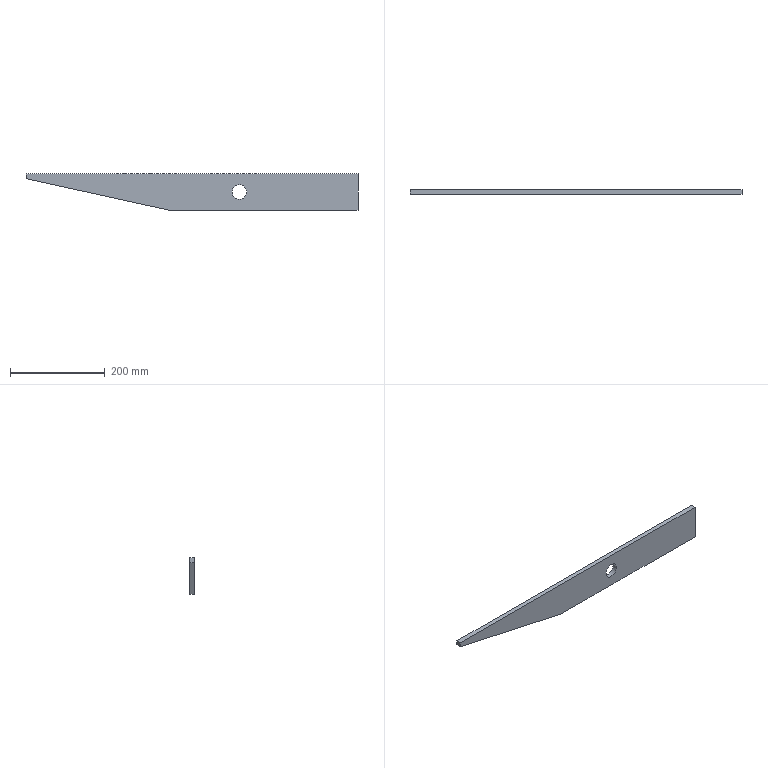Component | NX | CHAPA_FUNDO | 1 solid | 8 faces | box 700 x 10 x 76.2 mm | volume 426852 mm3 | plane 7 | cylinder 1 | commonest cylinder face diameters 31 x1
STEP:
#1=CARTESIAN_POINT('',(0.,0.,0.));
#2=DIRECTION('',(0.,0.,1.));
#3=DIRECTION('',(1.,0.,0.));
#4=AXIS2_PLACEMENT_3D('',#1,#2,#3);
#5=CARTESIAN_POINT('',(-60.,5.2,80.));
#6=VERTEX_POINT('',#5);
#7=CARTESIAN_POINT('',(-60.,5.2,3.8));
#8=VERTEX_POINT('',#7);
#9=CARTESIAN_POINT('',(-60.,5.2,80.));
#10=DIRECTION('',(-0.,0.,-1.));
#11=VECTOR('',#10,1.);
#12=LINE('',#9,#11);
#13=CARTESIAN_POINT('',(-60.,15.2,80.));
#14=DIRECTION('',(-1.,0.,0.));
#15=DIRECTION('',(-0.,0.,-1.));
#16=AXIS2_PLACEMENT_3D('',#13,#14,#15);
#17=PLANE('',#16);
#18=CARTESIAN_POINT('',(0.,10.));
#19=DIRECTION('',(1.,0.));
#20=VECTOR('',#19,1.);
#21=LINE('',#18,#20);
#22=(GEOMETRIC_REPRESENTATION_CONTEXT(2)PARAMETRIC_REPRESENTATION_CONTEXT()REPRESENTATION_CONTEXT('',''));
#23=DEFINITIONAL_REPRESENTATION('',(#21),#22);
#24=PCURVE('',#17,#23);
#25=CARTESIAN_POINT('',(-310.,5.2,41.9));
#26=DIRECTION('',(0.,1.,0.));
#27=DIRECTION('',(0.,0.,-1.));
#28=AXIS2_PLACEMENT_3D('',#25,#26,#27);
#29=PLANE('',#28);
#30=CARTESIAN_POINT('',(-38.1,-250.));
#31=DIRECTION('',(1.,0.));
#32=VECTOR('',#31,1.);
#33=LINE('',#30,#32);
#34=(GEOMETRIC_REPRESENTATION_CONTEXT(2)PARAMETRIC_REPRESENTATION_CONTEXT()REPRESENTATION_CONTEXT('',''));
#35=DEFINITIONAL_REPRESENTATION('',(#33),#34);
#36=PCURVE('',#29,#35);
#37=SURFACE_CURVE('',#12,(#24,#36),.PCURVE_S1.);
#38=EDGE_CURVE('',#6,#8,#37,.T.);
#39=ORIENTED_EDGE('',*,*,#38,.T.);
#40=CARTESIAN_POINT('',(-60.,15.2,3.8));
#41=VERTEX_POINT('',#40);
#42=CARTESIAN_POINT('',(-60.,15.2,3.8));
#43=DIRECTION('',(0.,-1.,0.));
#44=VECTOR('',#43,1.);
#45=LINE('',#42,#44);
#46=CARTESIAN_POINT('',(76.2,0.));
#47=DIRECTION('',(0.,1.));
#48=VECTOR('',#47,1.);
#49=LINE('',#46,#48);
#50=(GEOMETRIC_REPRESENTATION_CONTEXT(2)PARAMETRIC_REPRESENTATION_CONTEXT()REPRESENTATION_CONTEXT('',''));
#51=DEFINITIONAL_REPRESENTATION('',(#49),#50);
#52=PCURVE('',#17,#51);
#53=CARTESIAN_POINT('',(-60.,15.2,3.8));
#54=DIRECTION('',(0.,0.,1.));
#55=DIRECTION('',(-1.,0.,0.));
#56=AXIS2_PLACEMENT_3D('',#53,#54,#55);
#57=PLANE('',#56);
#58=CARTESIAN_POINT('',(0.,0.));
#59=DIRECTION('',(0.,1.));
#60=VECTOR('',#59,1.);
#61=LINE('',#58,#60);
#62=(GEOMETRIC_REPRESENTATION_CONTEXT(2)PARAMETRIC_REPRESENTATION_CONTEXT()REPRESENTATION_CONTEXT('',''));
#63=DEFINITIONAL_REPRESENTATION('',(#61),#62);
#64=PCURVE('',#57,#63);
#65=SURFACE_CURVE('',#45,(#52,#64),.PCURVE_S1.);
#66=EDGE_CURVE('',#41,#8,#65,.T.);
#67=ORIENTED_EDGE('',*,*,#66,.F.);
#68=CARTESIAN_POINT('',(-60.,15.2,80.));
#69=VERTEX_POINT('',#68);
#70=CARTESIAN_POINT('',(-60.,15.2,80.));
#71=DIRECTION('',(-0.,0.,-1.));
#72=VECTOR('',#71,1.);
#73=LINE('',#70,#72);
#74=CARTESIAN_POINT('',(0.,0.));
#75=DIRECTION('',(1.,0.));
#76=VECTOR('',#75,1.);
#77=LINE('',#74,#76);
#78=(GEOMETRIC_REPRESENTATION_CONTEXT(2)PARAMETRIC_REPRESENTATION_CONTEXT()REPRESENTATION_CONTEXT('',''));
#79=DEFINITIONAL_REPRESENTATION('',(#77),#78);
#80=PCURVE('',#17,#79);
#81=CARTESIAN_POINT('',(-310.,15.2,41.9));
#82=DIRECTION('',(0.,1.,0.));
#83=DIRECTION('',(0.,0.,-1.));
#84=AXIS2_PLACEMENT_3D('',#81,#82,#83);
#85=PLANE('',#84);
#86=CARTESIAN_POINT('',(-38.1,-250.));
#87=DIRECTION('',(1.,0.));
#88=VECTOR('',#87,1.);
#89=LINE('',#86,#88);
#90=(GEOMETRIC_REPRESENTATION_CONTEXT(2)PARAMETRIC_REPRESENTATION_CONTEXT()REPRESENTATION_CONTEXT('',''));
#91=DEFINITIONAL_REPRESENTATION('',(#89),#90);
#92=PCURVE('',#85,#91);
#93=SURFACE_CURVE('',#73,(#80,#92),.PCURVE_S1.);
#94=EDGE_CURVE('',#69,#41,#93,.T.);
#95=ORIENTED_EDGE('',*,*,#94,.F.);
#96=CARTESIAN_POINT('',(-60.,15.2,80.));
#97=DIRECTION('',(0.,-1.,0.));
#98=VECTOR('',#97,1.);
#99=LINE('',#96,#98);
#100=CARTESIAN_POINT('',(0.,0.));
#101=DIRECTION('',(0.,1.));
#102=VECTOR('',#101,1.);
#103=LINE('',#100,#102);
#104=(GEOMETRIC_REPRESENTATION_CONTEXT(2)PARAMETRIC_REPRESENTATION_CONTEXT()REPRESENTATION_CONTEXT('',''));
#105=DEFINITIONAL_REPRESENTATION('',(#103),#104);
#106=PCURVE('',#17,#105);
#107=CARTESIAN_POINT('',(-760.,15.2,80.));
#108=DIRECTION('',(-0.,0.,-1.));
#109=DIRECTION('',(1.,0.,-0.));
#110=AXIS2_PLACEMENT_3D('',#107,#108,#109);
#111=PLANE('',#110);
#112=CARTESIAN_POINT('',(700.,0.));
#113=DIRECTION('',(0.,1.));
#114=VECTOR('',#113,1.);
#115=LINE('',#112,#114);
#116=(GEOMETRIC_REPRESENTATION_CONTEXT(2)PARAMETRIC_REPRESENTATION_CONTEXT()REPRESENTATION_CONTEXT('',''));
#117=DEFINITIONAL_REPRESENTATION('',(#115),#116);
#118=PCURVE('',#111,#117);
#119=SURFACE_CURVE('',#99,(#106,#118),.PCURVE_S1.);
#120=EDGE_CURVE('',#69,#6,#119,.T.);
#121=ORIENTED_EDGE('',*,*,#120,.T.);
#122=EDGE_LOOP('',(#39,#67,#95,#121));
#123=FACE_BOUND('',#122,.T.);
#124=ADVANCED_FACE('',(#123),#17,.F.);
#125=CARTESIAN_POINT('',(-460.,5.2,3.8));
#126=VERTEX_POINT('',#125);
#127=CARTESIAN_POINT('',(-60.,5.2,3.8));
#128=DIRECTION('',(-1.,0.,0.));
#129=VECTOR('',#128,1.);
#130=LINE('',#127,#129);
#131=CARTESIAN_POINT('',(0.,10.));
#132=DIRECTION('',(1.,0.));
#133=VECTOR('',#132,1.);
#134=LINE('',#131,#133);
#135=(GEOMETRIC_REPRESENTATION_CONTEXT(2)PARAMETRIC_REPRESENTATION_CONTEXT()REPRESENTATION_CONTEXT('',''));
#136=DEFINITIONAL_REPRESENTATION('',(#134),#135);
#137=PCURVE('',#57,#136);
#138=CARTESIAN_POINT('',(38.1,-250.));
#139=DIRECTION('',(0.,1.));
#140=VECTOR('',#139,1.);
#141=LINE('',#138,#140);
#142=(GEOMETRIC_REPRESENTATION_CONTEXT(2)PARAMETRIC_REPRESENTATION_CONTEXT()REPRESENTATION_CONTEXT('',''));
#143=DEFINITIONAL_REPRESENTATION('',(#141),#142);
#144=PCURVE('',#29,#143);
#145=SURFACE_CURVE('',#130,(#137,#144),.PCURVE_S1.);
#146=EDGE_CURVE('',#8,#126,#145,.T.);
#147=ORIENTED_EDGE('',*,*,#146,.T.);
#148=CARTESIAN_POINT('',(-460.,15.2,3.8));
#149=VERTEX_POINT('',#148);
#150=CARTESIAN_POINT('',(-460.,15.2,3.8));
#151=DIRECTION('',(0.,-1.,0.));
#152=VECTOR('',#151,1.);
#153=LINE('',#150,#152);
#154=CARTESIAN_POINT('',(400.,0.));
#155=DIRECTION('',(0.,1.));
#156=VECTOR('',#155,1.);
#157=LINE('',#154,#156);
#158=(GEOMETRIC_REPRESENTATION_CONTEXT(2)PARAMETRIC_REPRESENTATION_CONTEXT()REPRESENTATION_CONTEXT('',''));
#159=DEFINITIONAL_REPRESENTATION('',(#157),#158);
#160=PCURVE('',#57,#159);
#161=CARTESIAN_POINT('',(-460.,15.2,3.8));
#162=DIRECTION('',(0.2149,0.,0.9766));
#163=DIRECTION('',(-0.9766,0.,0.2149));
#164=AXIS2_PLACEMENT_3D('',#161,#162,#163);
#165=PLANE('',#164);
#166=CARTESIAN_POINT('',(0.,0.));
#167=DIRECTION('',(0.,1.));
#168=VECTOR('',#167,1.);
#169=LINE('',#166,#168);
#170=(GEOMETRIC_REPRESENTATION_CONTEXT(2)PARAMETRIC_REPRESENTATION_CONTEXT()REPRESENTATION_CONTEXT('',''));
#171=DEFINITIONAL_REPRESENTATION('',(#169),#170);
#172=PCURVE('',#165,#171);
#173=SURFACE_CURVE('',#153,(#160,#172),.PCURVE_S1.);
#174=EDGE_CURVE('',#149,#126,#173,.T.);
#175=ORIENTED_EDGE('',*,*,#174,.F.);
#176=CARTESIAN_POINT('',(-60.,15.2,3.8));
#177=DIRECTION('',(-1.,0.,0.));
#178=VECTOR('',#177,1.);
#179=LINE('',#176,#178);
#180=CARTESIAN_POINT('',(0.,0.));
#181=DIRECTION('',(1.,0.));
#182=VECTOR('',#181,1.);
#183=LINE('',#180,#182);
#184=(GEOMETRIC_REPRESENTATION_CONTEXT(2)PARAMETRIC_REPRESENTATION_CONTEXT()REPRESENTATION_CONTEXT('',''));
#185=DEFINITIONAL_REPRESENTATION('',(#183),#184);
#186=PCURVE('',#57,#185);
#187=CARTESIAN_POINT('',(38.1,-250.));
#188=DIRECTION('',(0.,1.));
#189=VECTOR('',#188,1.);
#190=LINE('',#187,#189);
#191=(GEOMETRIC_REPRESENTATION_CONTEXT(2)PARAMETRIC_REPRESENTATION_CONTEXT()REPRESENTATION_CONTEXT('',''));
#192=DEFINITIONAL_REPRESENTATION('',(#190),#191);
#193=PCURVE('',#85,#192);
#194=SURFACE_CURVE('',#179,(#186,#193),.PCURVE_S1.);
#195=EDGE_CURVE('',#41,#149,#194,.T.);
#196=ORIENTED_EDGE('',*,*,#195,.F.);
#197=ORIENTED_EDGE('',*,*,#66,.T.);
#198=EDGE_LOOP('',(#147,#175,#196,#197));
#199=FACE_BOUND('',#198,.T.);
#200=ADVANCED_FACE('',(#199),#57,.F.);
#201=CARTESIAN_POINT('',(-760.,5.2,69.8));
#202=VERTEX_POINT('',#201);
#203=CARTESIAN_POINT('',(-460.,5.2,3.8));
#204=DIRECTION('',(-0.9766,0.,0.2149));
#205=VECTOR('',#204,1.);
#206=LINE('',#203,#205);
#207=CARTESIAN_POINT('',(0.,10.));
#208=DIRECTION('',(1.,0.));
#209=VECTOR('',#208,1.);
#210=LINE('',#207,#209);
#211=(GEOMETRIC_REPRESENTATION_CONTEXT(2)PARAMETRIC_REPRESENTATION_CONTEXT()REPRESENTATION_CONTEXT('',''));
#212=DEFINITIONAL_REPRESENTATION('',(#210),#211);
#213=PCURVE('',#165,#212);
#214=CARTESIAN_POINT('',(38.1,150.));
#215=DIRECTION('',(-0.2149,0.9766));
#216=VECTOR('',#215,1.);
#217=LINE('',#214,#216);
#218=(GEOMETRIC_REPRESENTATION_CONTEXT(2)PARAMETRIC_REPRESENTATION_CONTEXT()REPRESENTATION_CONTEXT('',''));
#219=DEFINITIONAL_REPRESENTATION('',(#217),#218);
#220=PCURVE('',#29,#219);
#221=SURFACE_CURVE('',#206,(#213,#220),.PCURVE_S1.);
#222=EDGE_CURVE('',#126,#202,#221,.T.);
#223=ORIENTED_EDGE('',*,*,#222,.T.);
#224=CARTESIAN_POINT('',(-760.,15.2,69.8));
#225=VERTEX_POINT('',#224);
#226=CARTESIAN_POINT('',(-760.,15.2,69.8));
#227=DIRECTION('',(0.,-1.,0.));
#228=VECTOR('',#227,1.);
#229=LINE('',#226,#228);
#230=CARTESIAN_POINT('',(307.174,0.));
#231=DIRECTION('',(0.,1.));
#232=VECTOR('',#231,1.);
#233=LINE('',#230,#232);
#234=(GEOMETRIC_REPRESENTATION_CONTEXT(2)PARAMETRIC_REPRESENTATION_CONTEXT()REPRESENTATION_CONTEXT('',''));
#235=DEFINITIONAL_REPRESENTATION('',(#233),#234);
#236=PCURVE('',#165,#235);
#237=CARTESIAN_POINT('',(-760.,15.2,69.8));
#238=DIRECTION('',(1.,0.,0.));
#239=DIRECTION('',(0.,0.,1.));
#240=AXIS2_PLACEMENT_3D('',#237,#238,#239);
#241=PLANE('',#240);
#242=CARTESIAN_POINT('',(0.,0.));
#243=DIRECTION('',(0.,1.));
#244=VECTOR('',#243,1.);
#245=LINE('',#242,#244);
#246=(GEOMETRIC_REPRESENTATION_CONTEXT(2)PARAMETRIC_REPRESENTATION_CONTEXT()REPRESENTATION_CONTEXT('',''));
#247=DEFINITIONAL_REPRESENTATION('',(#245),#246);
#248=PCURVE('',#241,#247);
#249=SURFACE_CURVE('',#229,(#236,#248),.PCURVE_S1.);
#250=EDGE_CURVE('',#225,#202,#249,.T.);
#251=ORIENTED_EDGE('',*,*,#250,.F.);
#252=CARTESIAN_POINT('',(-460.,15.2,3.8));
#253=DIRECTION('',(-0.9766,0.,0.2149));
#254=VECTOR('',#253,1.);
#255=LINE('',#252,#254);
#256=CARTESIAN_POINT('',(0.,0.));
#257=DIRECTION('',(1.,0.));
#258=VECTOR('',#257,1.);
#259=LINE('',#256,#258);
#260=(GEOMETRIC_REPRESENTATION_CONTEXT(2)PARAMETRIC_REPRESENTATION_CONTEXT()REPRESENTATION_CONTEXT('',''));
#261=DEFINITIONAL_REPRESENTATION('',(#259),#260);
#262=PCURVE('',#165,#261);
#263=CARTESIAN_POINT('',(38.1,150.));
#264=DIRECTION('',(-0.2149,0.9766));
#265=VECTOR('',#264,1.);
#266=LINE('',#263,#265);
#267=(GEOMETRIC_REPRESENTATION_CONTEXT(2)PARAMETRIC_REPRESENTATION_CONTEXT()REPRESENTATION_CONTEXT('',''));
#268=DEFINITIONAL_REPRESENTATION('',(#266),#267);
#269=PCURVE('',#85,#268);
#270=SURFACE_CURVE('',#255,(#262,#269),.PCURVE_S1.);
#271=EDGE_CURVE('',#149,#225,#270,.T.);
#272=ORIENTED_EDGE('',*,*,#271,.F.);
#273=ORIENTED_EDGE('',*,*,#174,.T.);
#274=EDGE_LOOP('',(#223,#251,#272,#273));
#275=FACE_BOUND('',#274,.T.);
#276=ADVANCED_FACE('',(#275),#165,.F.);
#277=CARTESIAN_POINT('',(-760.,5.2,80.));
#278=VERTEX_POINT('',#277);
#279=CARTESIAN_POINT('',(-760.,5.2,69.8));
#280=DIRECTION('',(0.,0.,1.));
#281=VECTOR('',#280,1.);
#282=LINE('',#279,#281);
#283=CARTESIAN_POINT('',(0.,10.));
#284=DIRECTION('',(1.,0.));
#285=VECTOR('',#284,1.);
#286=LINE('',#283,#285);
#287=(GEOMETRIC_REPRESENTATION_CONTEXT(2)PARAMETRIC_REPRESENTATION_CONTEXT()REPRESENTATION_CONTEXT('',''));
#288=DEFINITIONAL_REPRESENTATION('',(#286),#287);
#289=PCURVE('',#241,#288);
#290=CARTESIAN_POINT('',(-27.9,450.));
#291=DIRECTION('',(-1.,0.));
#292=VECTOR('',#291,1.);
#293=LINE('',#290,#292);
#294=(GEOMETRIC_REPRESENTATION_CONTEXT(2)PARAMETRIC_REPRESENTATION_CONTEXT()REPRESENTATION_CONTEXT('',''));
#295=DEFINITIONAL_REPRESENTATION('',(#293),#294);
#296=PCURVE('',#29,#295);
#297=SURFACE_CURVE('',#282,(#289,#296),.PCURVE_S1.);
#298=EDGE_CURVE('',#202,#278,#297,.T.);
#299=ORIENTED_EDGE('',*,*,#298,.T.);
#300=CARTESIAN_POINT('',(-760.,15.2,80.));
#301=VERTEX_POINT('',#300);
#302=CARTESIAN_POINT('',(-760.,15.2,80.));
#303=DIRECTION('',(0.,-1.,0.));
#304=VECTOR('',#303,1.);
#305=LINE('',#302,#304);
#306=CARTESIAN_POINT('',(10.2,0.));
#307=DIRECTION('',(0.,1.));
#308=VECTOR('',#307,1.);
#309=LINE('',#306,#308);
#310=(GEOMETRIC_REPRESENTATION_CONTEXT(2)PARAMETRIC_REPRESENTATION_CONTEXT()REPRESENTATION_CONTEXT('',''));
#311=DEFINITIONAL_REPRESENTATION('',(#309),#310);
#312=PCURVE('',#241,#311);
#313=CARTESIAN_POINT('',(0.,0.));
#314=DIRECTION('',(0.,1.));
#315=VECTOR('',#314,1.);
#316=LINE('',#313,#315);
#317=(GEOMETRIC_REPRESENTATION_CONTEXT(2)PARAMETRIC_REPRESENTATION_CONTEXT()REPRESENTATION_CONTEXT('',''));
#318=DEFINITIONAL_REPRESENTATION('',(#316),#317);
#319=PCURVE('',#111,#318);
#320=SURFACE_CURVE('',#305,(#312,#319),.PCURVE_S1.);
#321=EDGE_CURVE('',#301,#278,#320,.T.);
#322=ORIENTED_EDGE('',*,*,#321,.F.);
#323=CARTESIAN_POINT('',(-760.,15.2,69.8));
#324=DIRECTION('',(0.,0.,1.));
#325=VECTOR('',#324,1.);
#326=LINE('',#323,#325);
#327=CARTESIAN_POINT('',(0.,0.));
#328=DIRECTION('',(1.,0.));
#329=VECTOR('',#328,1.);
#330=LINE('',#327,#329);
#331=(GEOMETRIC_REPRESENTATION_CONTEXT(2)PARAMETRIC_REPRESENTATION_CONTEXT()REPRESENTATION_CONTEXT('',''));
#332=DEFINITIONAL_REPRESENTATION('',(#330),#331);
#333=PCURVE('',#241,#332);
#334=CARTESIAN_POINT('',(-27.9,450.));
#335=DIRECTION('',(-1.,0.));
#336=VECTOR('',#335,1.);
#337=LINE('',#334,#336);
#338=(GEOMETRIC_REPRESENTATION_CONTEXT(2)PARAMETRIC_REPRESENTATION_CONTEXT()REPRESENTATION_CONTEXT('',''));
#339=DEFINITIONAL_REPRESENTATION('',(#337),#338);
#340=PCURVE('',#85,#339);
#341=SURFACE_CURVE('',#326,(#333,#340),.PCURVE_S1.);
#342=EDGE_CURVE('',#225,#301,#341,.T.);
#343=ORIENTED_EDGE('',*,*,#342,.F.);
#344=ORIENTED_EDGE('',*,*,#250,.T.);
#345=EDGE_LOOP('',(#299,#322,#343,#344));
#346=FACE_BOUND('',#345,.T.);
#347=ADVANCED_FACE('',(#346),#241,.F.);
#348=CARTESIAN_POINT('',(-760.,5.2,80.));
#349=DIRECTION('',(1.,0.,-0.));
#350=VECTOR('',#349,1.);
#351=LINE('',#348,#350);
#352=CARTESIAN_POINT('',(0.,10.));
#353=DIRECTION('',(1.,0.));
#354=VECTOR('',#353,1.);
#355=LINE('',#352,#354);
#356=(GEOMETRIC_REPRESENTATION_CONTEXT(2)PARAMETRIC_REPRESENTATION_CONTEXT()REPRESENTATION_CONTEXT('',''));
#357=DEFINITIONAL_REPRESENTATION('',(#355),#356);
#358=PCURVE('',#111,#357);
#359=CARTESIAN_POINT('',(-38.1,450.));
#360=DIRECTION('',(0.,-1.));
#361=VECTOR('',#360,1.);
#362=LINE('',#359,#361);
#363=(GEOMETRIC_REPRESENTATION_CONTEXT(2)PARAMETRIC_REPRESENTATION_CONTEXT()REPRESENTATION_CONTEXT('',''));
#364=DEFINITIONAL_REPRESENTATION('',(#362),#363);
#365=PCURVE('',#29,#364);
#366=SURFACE_CURVE('',#351,(#358,#365),.PCURVE_S1.);
#367=EDGE_CURVE('',#278,#6,#366,.T.);
#368=ORIENTED_EDGE('',*,*,#367,.T.);
#369=ORIENTED_EDGE('',*,*,#120,.F.);
#370=CARTESIAN_POINT('',(-760.,15.2,80.));
#371=DIRECTION('',(1.,0.,-0.));
#372=VECTOR('',#371,1.);
#373=LINE('',#370,#372);
#374=CARTESIAN_POINT('',(0.,0.));
#375=DIRECTION('',(1.,0.));
#376=VECTOR('',#375,1.);
#377=LINE('',#374,#376);
#378=(GEOMETRIC_REPRESENTATION_CONTEXT(2)PARAMETRIC_REPRESENTATION_CONTEXT()REPRESENTATION_CONTEXT('',''));
#379=DEFINITIONAL_REPRESENTATION('',(#377),#378);
#380=PCURVE('',#111,#379);
#381=CARTESIAN_POINT('',(-38.1,450.));
#382=DIRECTION('',(0.,-1.));
#383=VECTOR('',#382,1.);
#384=LINE('',#381,#383);
#385=(GEOMETRIC_REPRESENTATION_CONTEXT(2)PARAMETRIC_REPRESENTATION_CONTEXT()REPRESENTATION_CONTEXT('',''));
#386=DEFINITIONAL_REPRESENTATION('',(#384),#385);
#387=PCURVE('',#85,#386);
#388=SURFACE_CURVE('',#373,(#380,#387),.PCURVE_S1.);
#389=EDGE_CURVE('',#301,#69,#388,.T.);
#390=ORIENTED_EDGE('',*,*,#389,.F.);
#391=ORIENTED_EDGE('',*,*,#321,.T.);
#392=EDGE_LOOP('',(#368,#369,#390,#391));
#393=FACE_BOUND('',#392,.T.);
#394=ADVANCED_FACE('',(#393),#111,.F.);
#395=CARTESIAN_POINT('',(-325.5,15.2,41.9));
#396=VERTEX_POINT('',#395);
#397=CARTESIAN_POINT('',(-310.,15.2,41.9));
#398=DIRECTION('',(0.,1.,0.));
#399=DIRECTION('',(-1.,0.,0.));
#400=AXIS2_PLACEMENT_3D('',#397,#398,#399);
#401=CIRCLE('',#400,15.5);
#402=CARTESIAN_POINT('',(-310.,15.2,41.9));
#403=DIRECTION('',(0.,-1.,0.));
#404=DIRECTION('',(0.,0.,1.));
#405=AXIS2_PLACEMENT_3D('',#402,#403,#404);
#406=CYLINDRICAL_SURFACE('',#405,15.5);
#407=CARTESIAN_POINT('',(7.854,0.));
#408=DIRECTION('',(-1.,0.));
#409=VECTOR('',#408,1.);
#410=LINE('',#407,#409);
#411=(GEOMETRIC_REPRESENTATION_CONTEXT(2)PARAMETRIC_REPRESENTATION_CONTEXT()REPRESENTATION_CONTEXT('',''));
#412=DEFINITIONAL_REPRESENTATION('',(#410),#411);
#413=PCURVE('',#406,#412);
#414=CARTESIAN_POINT('',(0.,0.));
#415=DIRECTION('',(0.,1.));
#416=AXIS2_PLACEMENT_2D('',#414,#415);
#417=CIRCLE('',#416,15.5);
#418=(GEOMETRIC_REPRESENTATION_CONTEXT(2)PARAMETRIC_REPRESENTATION_CONTEXT()REPRESENTATION_CONTEXT('',''));
#419=DEFINITIONAL_REPRESENTATION('',(#417),#418);
#420=PCURVE('',#85,#419);
#421=SURFACE_CURVE('',#401,(#413,#420),.PCURVE_S1.);
#422=EDGE_CURVE('',#396,#396,#421,.T.);
#423=ORIENTED_EDGE('',*,*,#422,.F.);
#424=CARTESIAN_POINT('',(-325.5,5.2,41.9));
#425=VERTEX_POINT('',#424);
#426=CARTESIAN_POINT('',(-325.5,15.2,41.9));
#427=CARTESIAN_POINT('',(-325.5,5.2,41.9));
#428=B_SPLINE_CURVE_WITH_KNOTS('',1,(#426,#427),.UNSPECIFIED.,.F.,.F.,(2,2),(0.,10.),.PIECEWISE_BEZIER_KNOTS.);
#429=CARTESIAN_POINT('',(7.854,0.));
#430=DIRECTION('',(0.,1.));
#431=VECTOR('',#430,1.);
#432=LINE('',#429,#431);
#433=(GEOMETRIC_REPRESENTATION_CONTEXT(2)PARAMETRIC_REPRESENTATION_CONTEXT()REPRESENTATION_CONTEXT('',''));
#434=DEFINITIONAL_REPRESENTATION('',(#432),#433);
#435=PCURVE('',#406,#434);
#436=CARTESIAN_POINT('',(1.571,0.));
#437=DIRECTION('',(0.,1.));
#438=VECTOR('',#437,1.);
#439=LINE('',#436,#438);
#440=(GEOMETRIC_REPRESENTATION_CONTEXT(2)PARAMETRIC_REPRESENTATION_CONTEXT()REPRESENTATION_CONTEXT('',''));
#441=DEFINITIONAL_REPRESENTATION('',(#439),#440);
#442=PCURVE('',#406,#441);
#443=SEAM_CURVE('',#428,(#435,#442),.PCURVE_S1.);
#444=EDGE_CURVE('',#396,#425,#443,.T.);
#445=ORIENTED_EDGE('',*,*,#444,.T.);
#446=CARTESIAN_POINT('',(-310.,5.2,41.9));
#447=DIRECTION('',(0.,1.,0.));
#448=DIRECTION('',(-1.,0.,0.));
#449=AXIS2_PLACEMENT_3D('',#446,#447,#448);
#450=CIRCLE('',#449,15.5);
#451=CARTESIAN_POINT('',(7.854,10.));
#452=DIRECTION('',(-1.,0.));
#453=VECTOR('',#452,1.);
#454=LINE('',#451,#453);
#455=(GEOMETRIC_REPRESENTATION_CONTEXT(2)PARAMETRIC_REPRESENTATION_CONTEXT()REPRESENTATION_CONTEXT('',''));
#456=DEFINITIONAL_REPRESENTATION('',(#454),#455);
#457=PCURVE('',#406,#456);
#458=CARTESIAN_POINT('',(0.,0.));
#459=DIRECTION('',(0.,1.));
#460=AXIS2_PLACEMENT_2D('',#458,#459);
#461=CIRCLE('',#460,15.5);
#462=(GEOMETRIC_REPRESENTATION_CONTEXT(2)PARAMETRIC_REPRESENTATION_CONTEXT()REPRESENTATION_CONTEXT('',''));
#463=DEFINITIONAL_REPRESENTATION('',(#461),#462);
#464=PCURVE('',#29,#463);
#465=SURFACE_CURVE('',#450,(#457,#464),.PCURVE_S1.);
#466=EDGE_CURVE('',#425,#425,#465,.T.);
#467=ORIENTED_EDGE('',*,*,#466,.T.);
#468=ORIENTED_EDGE('',*,*,#444,.F.);
#469=EDGE_LOOP('',(#423,#445,#467,#468));
#470=FACE_BOUND('',#469,.F.);
#471=ADVANCED_FACE('',(#470),#406,.F.);
#472=ORIENTED_EDGE('',*,*,#94,.T.);
#473=ORIENTED_EDGE('',*,*,#195,.T.);
#474=ORIENTED_EDGE('',*,*,#271,.T.);
#475=ORIENTED_EDGE('',*,*,#342,.T.);
#476=ORIENTED_EDGE('',*,*,#389,.T.);
#477=EDGE_LOOP('',(#472,#473,#474,#475,#476));
#478=FACE_BOUND('',#477,.T.);
#479=ORIENTED_EDGE('',*,*,#422,.F.);
#480=EDGE_LOOP('',(#479));
#481=FACE_BOUND('',#480,.T.);
#482=ADVANCED_FACE('',(#478,#481),#85,.T.);
#483=ORIENTED_EDGE('',*,*,#38,.F.);
#484=ORIENTED_EDGE('',*,*,#367,.F.);
#485=ORIENTED_EDGE('',*,*,#298,.F.);
#486=ORIENTED_EDGE('',*,*,#222,.F.);
#487=ORIENTED_EDGE('',*,*,#146,.F.);
#488=EDGE_LOOP('',(#483,#484,#485,#486,#487));
#489=FACE_BOUND('',#488,.T.);
#490=ORIENTED_EDGE('',*,*,#466,.T.);
#491=EDGE_LOOP('',(#490));
#492=FACE_BOUND('',#491,.T.);
#493=ADVANCED_FACE('',(#489,#492),#29,.F.);
#494=CLOSED_SHELL('',(#124,#200,#276,#347,#394,#471,#482,#493));
#495=MANIFOLD_SOLID_BREP('',#494);
#496=(LENGTH_UNIT()NAMED_UNIT(*)SI_UNIT(.MILLI.,.METRE.));
#497=UNCERTAINTY_MEASURE_WITH_UNIT(LENGTH_MEASURE(0.000001),#496,'','');
#498=(NAMED_UNIT(*)PLANE_ANGLE_UNIT()SI_UNIT($,.RADIAN.));
#499=(NAMED_UNIT(*)SI_UNIT($,.STERADIAN.)SOLID_ANGLE_UNIT());
#500=(GEOMETRIC_REPRESENTATION_CONTEXT(3)GLOBAL_UNCERTAINTY_ASSIGNED_CONTEXT((#497))GLOBAL_UNIT_ASSIGNED_CONTEXT((#496,#498,#499))REPRESENTATION_CONTEXT('',''));
#501=ADVANCED_BREP_SHAPE_REPRESENTATION('',(#4,#495),#500);